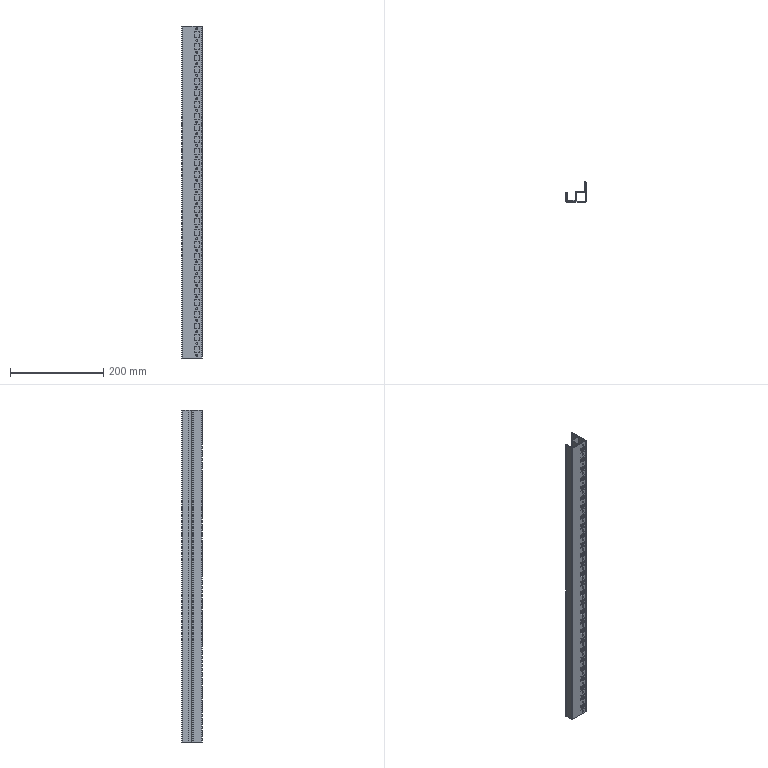Component | SolidWorks | CabinetFrameWeldmentDrawingPG50-01-00-1_FrontAndRearBeamPG50-01-105-1 | 1 solid | 382 faces | volume 205419 mm3 | plane 248 | cylinder 134 | commonest cylinder face diameters 4.1 x116 1 x8 3.999 x6 4 x2 0.02 x1 3 x1 | material AISI 1045 Steel, cold drawn